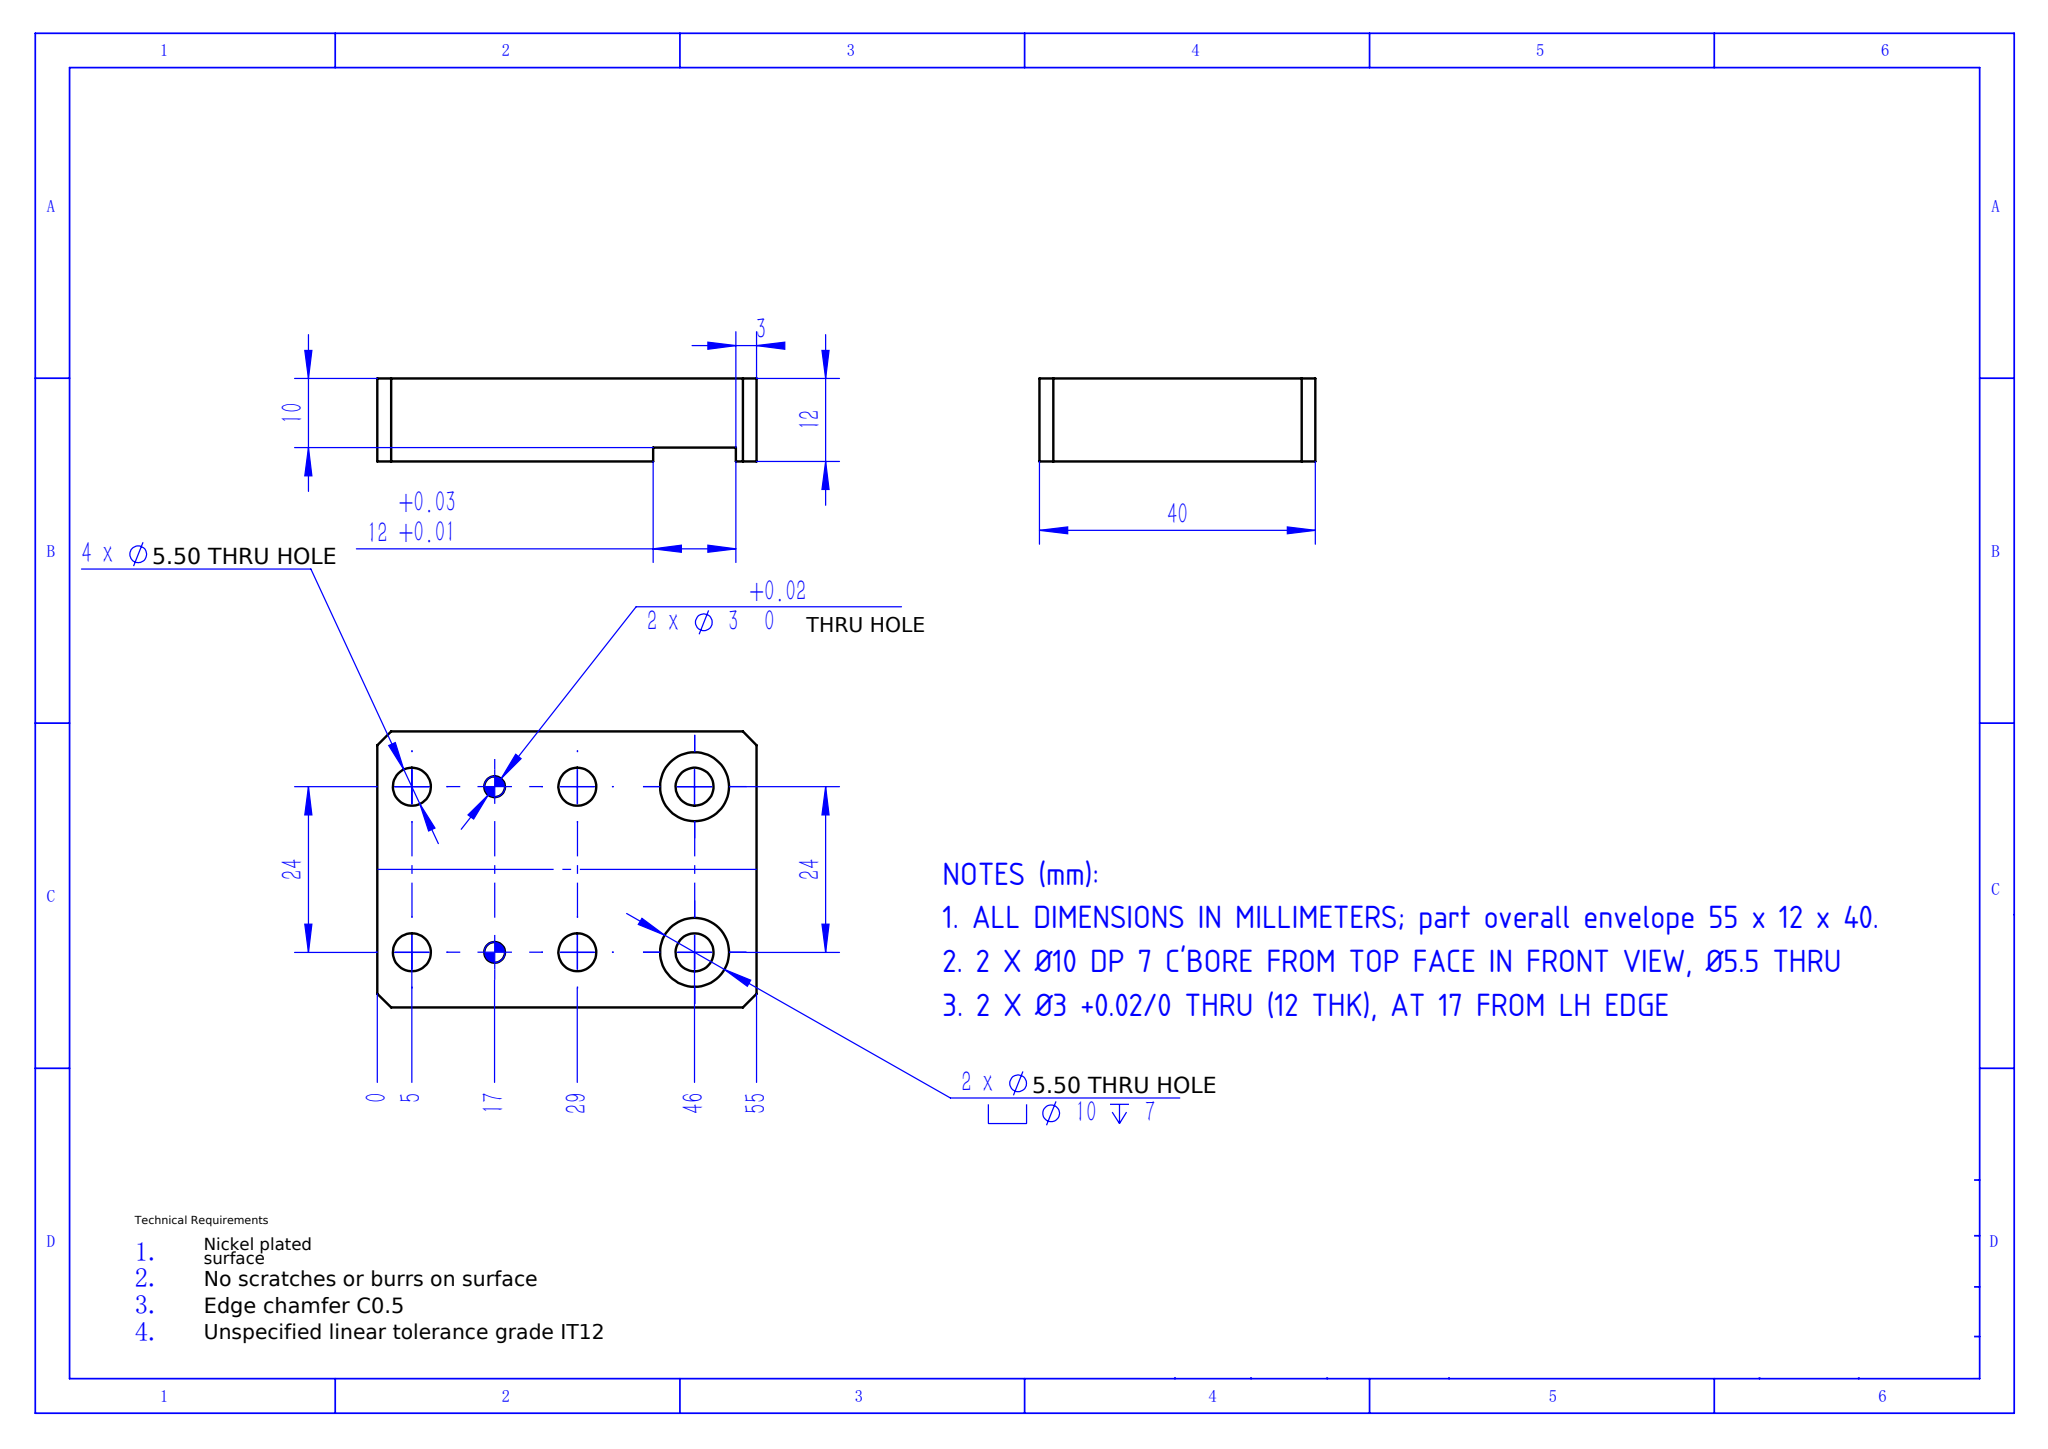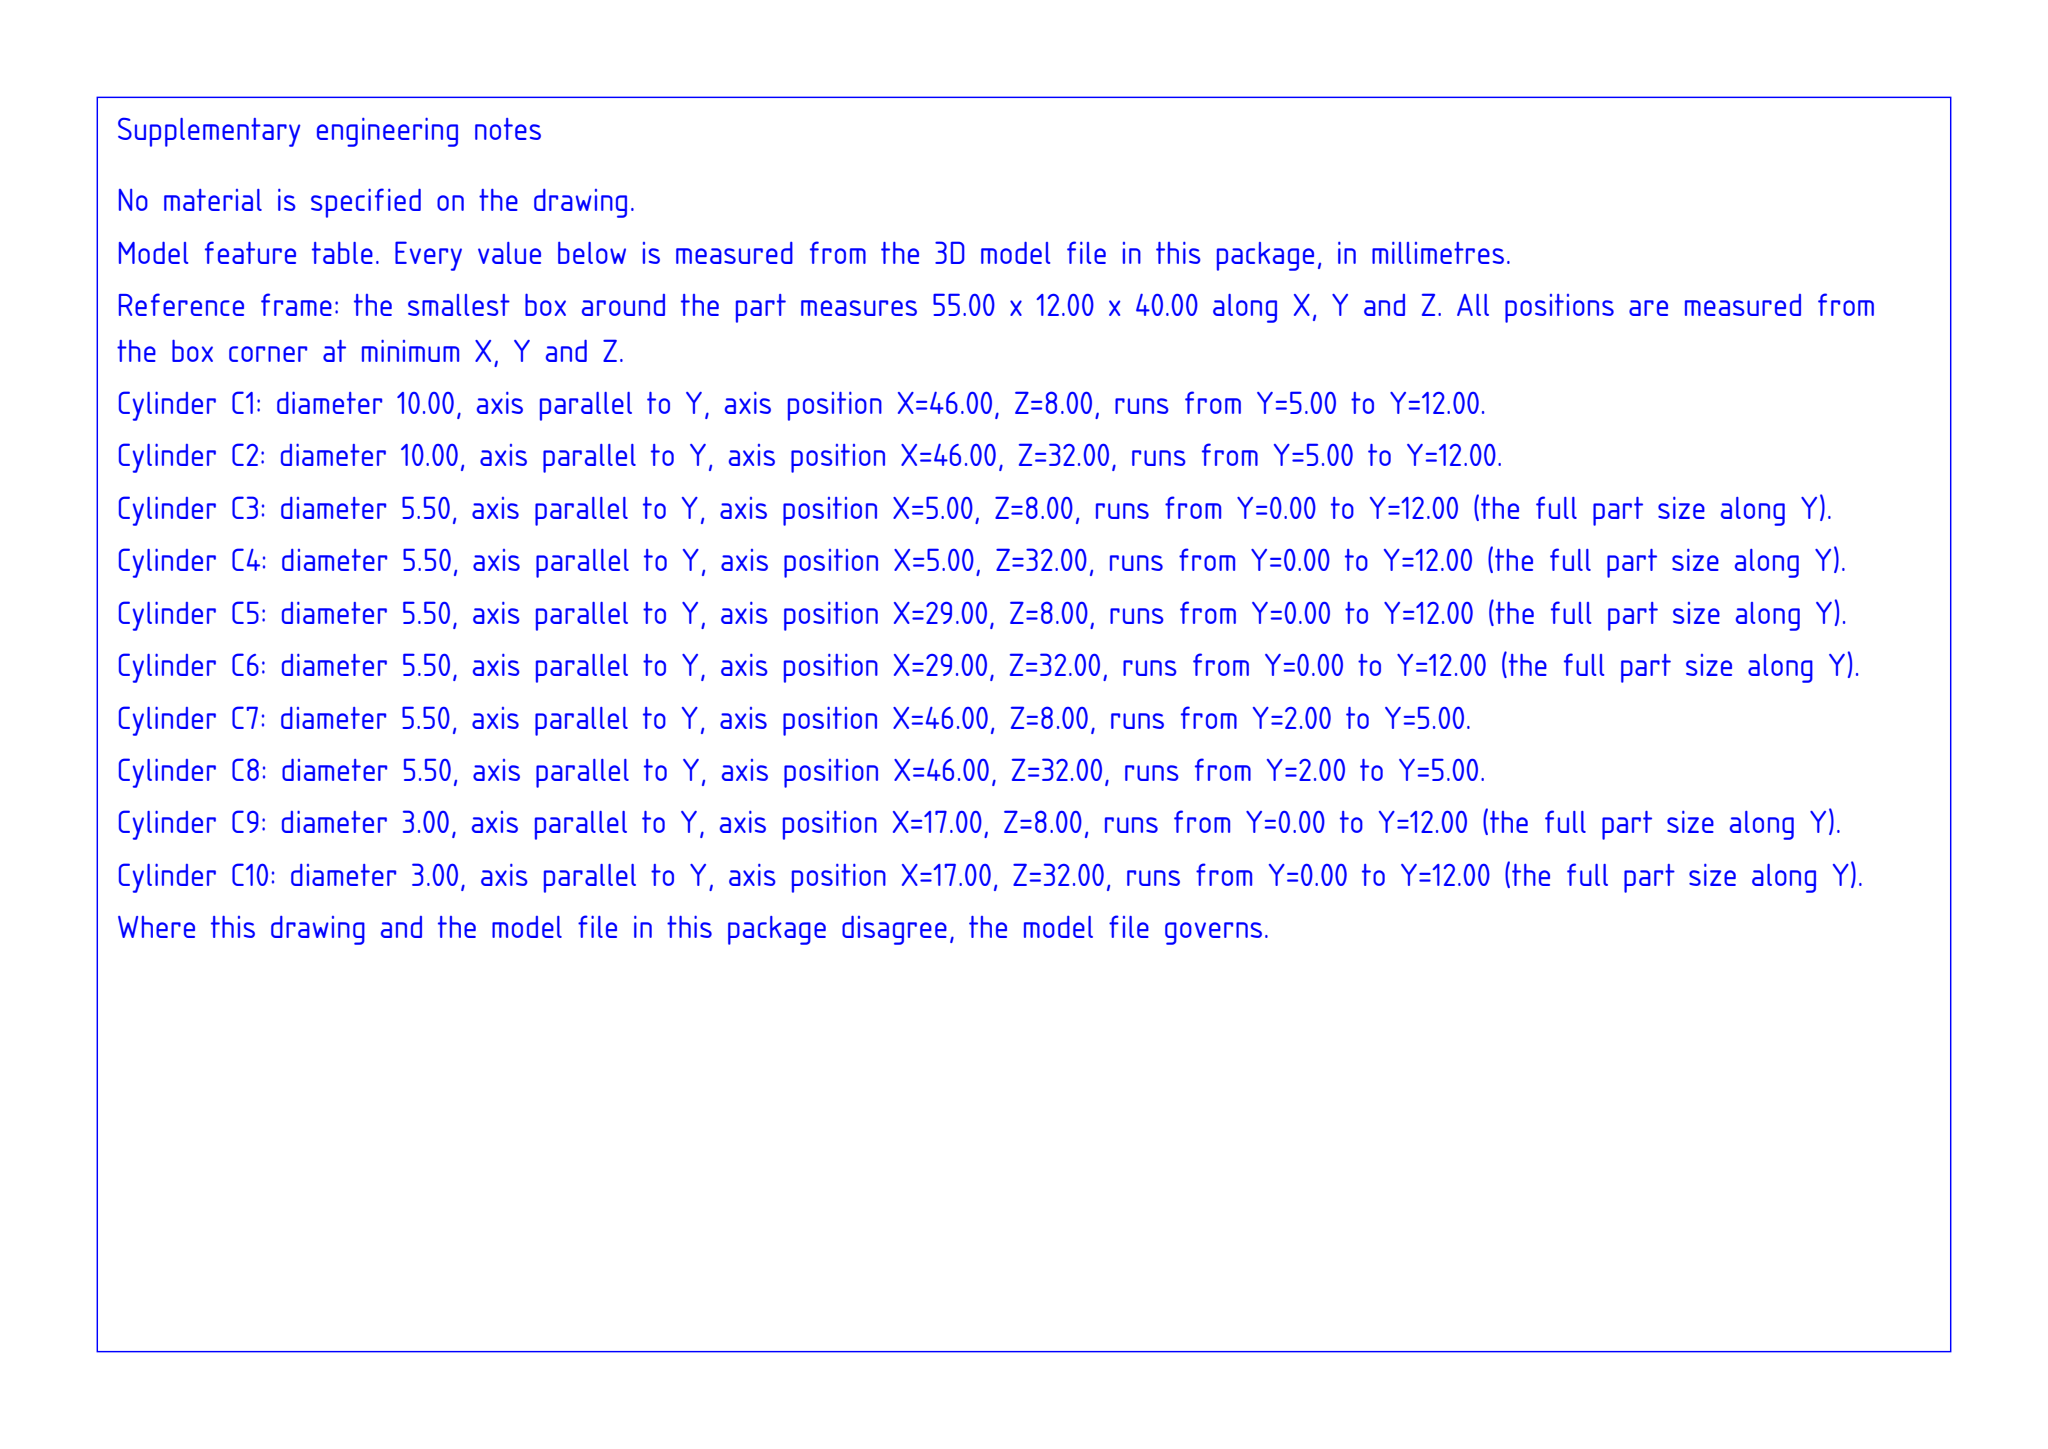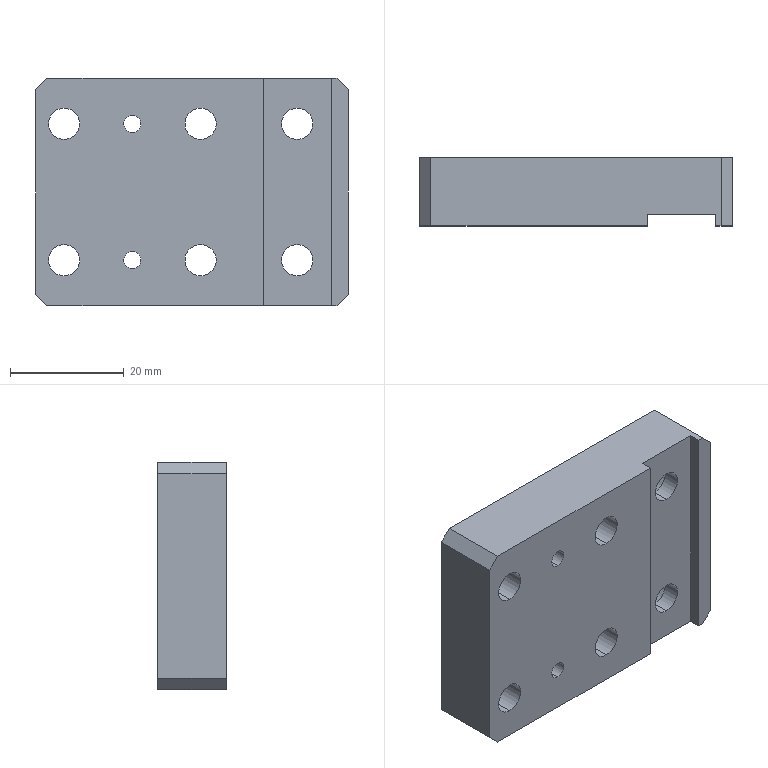Part | SolidWorks | mm | 1 solid | 36 faces | box 55 x 12 x 40 mm | volume 22792 mm3 | cylinder 20 | plane 16 | commonest cylinder face diameters 5.5 x12 10 x4 3 x4
Drawing notes:
ALL DIMENSIONS IN MILLIMETERS; part overall envelope 55 x 12 x 40. | from the solid: bbox_xyz [55.0, 12.0, 40.0] in mm
2 X Ø10 DP 7 C'BORE FROM TOP FACE IN FRONT VIEW, Ø5.5 THRU | from the solid: Ø10 cyl at x=46, z=8 & 32, len 7 from y=12 face; Ø5.5 len 3 to y=2; c'bore bottoms = planes y=5 (2); part y 2..12 = 10 thk at that area
2 X Ø3 +0.02/0 THRU (12 THK), AT 17 FROM LH EDGE | from the solid: cylinders [3.0,'y',[17.0,null,8.0],12.0] and [3.0,'y',[17.0,null,32.0],12.0]; full 12 mm thickness = THRU
build123d program:
from build123d import *

# Parameters (mm, degrees)
SKETCH1_W                                         = 55
SKETCH1_H                                         = 40
BOSS_EXTRUDE1_DEPTH                               = 12
M5_CLEARANCE_HOLE1_D                              = 5.5
SIZE_MM_DOWEL_PIN_HOLE1_D                         = 3
SKETCH6_W                                         = 12
SKETCH6_H                                         = 40
CUT_EXTRUDE1_DEPTH                                = 2
HOLE_SIZE_ACCORDING_TO_HEX_SOCKET_HEA_D           = 5.5
HOLE_SIZE_ACCORDING_TO_HEX_SOCKET_HEA_CBORE_D     = 10
HOLE_SIZE_ACCORDING_TO_HEX_SOCKET_HEA_CBORE_DEPTH = 7
CHAMFER1_SIZE                                     = 2


with BuildPart() as part:
    # Sketch1 → Boss-Extrude1 (new body)
    with BuildSketch(Plane(origin=(0, 0, 0), x_dir=(1, 0, 0), z_dir=(0, 1, 0))):
        with Locations((27.5, 0)):
            Rectangle(SKETCH1_W, SKETCH1_H)
    extrude(amount=BOSS_EXTRUDE1_DEPTH)

    # M5 Clearance Hole1 (through all)
    with Locations(Plane(origin=(0, 0, 0), x_dir=(-1, 0, 0), z_dir=(0, -1, 0))):
        with Locations((-5, 12), (-5, -12), (-29, -12), (-29, 12)):
            Hole(M5_CLEARANCE_HOLE1_D / 2)

    # Size mm Dowel Pin Hole1 (through all)
    with Locations(Plane(origin=(0, 0, 0), x_dir=(-1, 0, 0), z_dir=(0, -1, 0))):
        with Locations((-17, 12), (-17, -12)):
            Hole(SIZE_MM_DOWEL_PIN_HOLE1_D / 2)

    # Sketch6 → Cut-Extrude1 (cut)
    with BuildSketch(Plane.XZ):
        with Locations((46, 0)):
            Rectangle(SKETCH6_W, SKETCH6_H)
    extrude(amount=-CUT_EXTRUDE1_DEPTH, mode=Mode.SUBTRACT)

    # Hole Size _ according to_ Hex Socket Hea (through all)
    with Locations(Plane(origin=(0, 12, 0), x_dir=(1, 0, 0), z_dir=(0, 1, 0))):
        with Locations((46, 12), (46, -12)):
            CounterBoreHole(HOLE_SIZE_ACCORDING_TO_HEX_SOCKET_HEA_D / 2, HOLE_SIZE_ACCORDING_TO_HEX_SOCKET_HEA_CBORE_D / 2, HOLE_SIZE_ACCORDING_TO_HEX_SOCKET_HEA_CBORE_DEPTH)

    # Chamfer1
    chamfer1_edges = [part.edges().sort_by_distance(p)[0] for p in [
        (0, 6, -20),
        (55, 6, -20),
        (55, 6, 20),
        (0, 6, 20),
    ]]
    chamfer(chamfer1_edges, length=CHAMFER1_SIZE)


solid = part.part